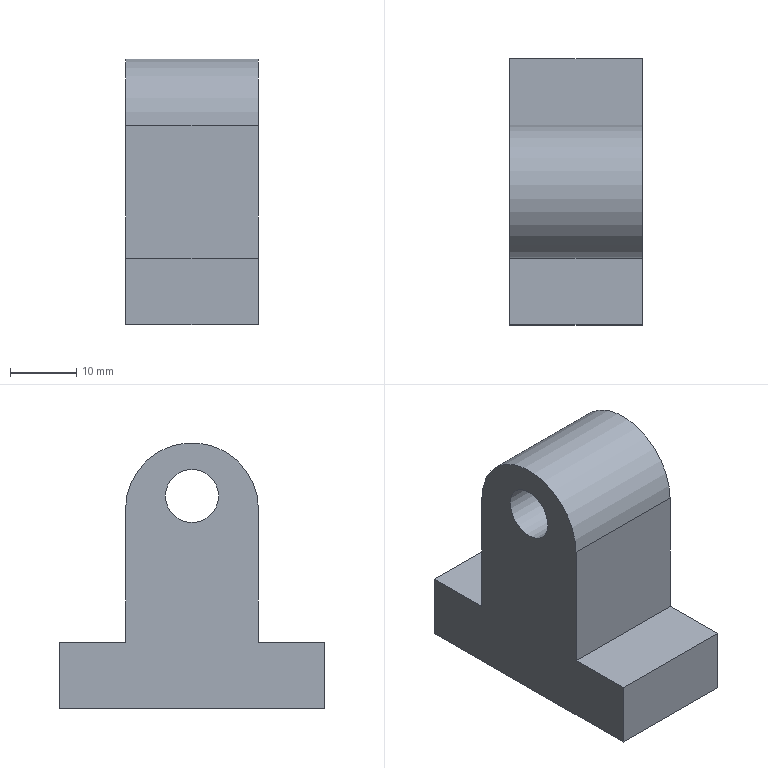Component | NX | T_SLIDER | 1 solid | 11 faces | box 20 x 40 x 40 mm | volume 18136 mm3 | plane 9 | cylinder 2 | commonest cylinder face diameters 20 x1 8 x1
STEP:
#1=CARTESIAN_POINT('',(0.,0.,0.));
#2=DIRECTION('',(0.,0.,1.));
#3=DIRECTION('',(1.,0.,0.));
#4=AXIS2_PLACEMENT_3D('',#1,#2,#3);
#5=CARTESIAN_POINT('',(-4.,-20.,10.));
#6=VERTEX_POINT('',#5);
#7=CARTESIAN_POINT('',(-4.,-20.,0.));
#8=VERTEX_POINT('',#7);
#9=CARTESIAN_POINT('',(-4.,-20.,10.));
#10=DIRECTION('',(0.,0.,-1.));
#11=VECTOR('',#10,1.);
#12=LINE('',#9,#11);
#13=CARTESIAN_POINT('',(16.,-20.,10.));
#14=DIRECTION('',(0.,1.,0.));
#15=DIRECTION('',(0.,-0.,1.));
#16=AXIS2_PLACEMENT_3D('',#13,#14,#15);
#17=PLANE('',#16);
#18=CARTESIAN_POINT('',(0.,-20.));
#19=DIRECTION('',(-1.,0.));
#20=VECTOR('',#19,1.);
#21=LINE('',#18,#20);
#22=(GEOMETRIC_REPRESENTATION_CONTEXT(2)PARAMETRIC_REPRESENTATION_CONTEXT()REPRESENTATION_CONTEXT('',''));
#23=DEFINITIONAL_REPRESENTATION('',(#21),#22);
#24=PCURVE('',#17,#23);
#25=CARTESIAN_POINT('',(-4.,-0.,30.));
#26=DIRECTION('',(1.,0.,0.));
#27=DIRECTION('',(0.,0.,-1.));
#28=AXIS2_PLACEMENT_3D('',#25,#26,#27);
#29=PLANE('',#28);
#30=CARTESIAN_POINT('',(20.,-20.));
#31=DIRECTION('',(1.,0.));
#32=VECTOR('',#31,1.);
#33=LINE('',#30,#32);
#34=(GEOMETRIC_REPRESENTATION_CONTEXT(2)PARAMETRIC_REPRESENTATION_CONTEXT()REPRESENTATION_CONTEXT('',''));
#35=DEFINITIONAL_REPRESENTATION('',(#33),#34);
#36=PCURVE('',#29,#35);
#37=SURFACE_CURVE('',#12,(#24,#36),.PCURVE_S1.);
#38=EDGE_CURVE('',#6,#8,#37,.T.);
#39=ORIENTED_EDGE('',*,*,#38,.T.);
#40=CARTESIAN_POINT('',(16.,-20.,0.));
#41=VERTEX_POINT('',#40);
#42=CARTESIAN_POINT('',(16.,-20.,0.));
#43=DIRECTION('',(-1.,0.,0.));
#44=VECTOR('',#43,1.);
#45=LINE('',#42,#44);
#46=CARTESIAN_POINT('',(-10.,0.));
#47=DIRECTION('',(0.,-1.));
#48=VECTOR('',#47,1.);
#49=LINE('',#46,#48);
#50=(GEOMETRIC_REPRESENTATION_CONTEXT(2)PARAMETRIC_REPRESENTATION_CONTEXT()REPRESENTATION_CONTEXT('',''));
#51=DEFINITIONAL_REPRESENTATION('',(#49),#50);
#52=PCURVE('',#17,#51);
#53=CARTESIAN_POINT('',(16.,-20.,0.));
#54=DIRECTION('',(0.,0.,1.));
#55=DIRECTION('',(1.,0.,0.));
#56=AXIS2_PLACEMENT_3D('',#53,#54,#55);
#57=PLANE('',#56);
#58=CARTESIAN_POINT('',(0.,0.));
#59=DIRECTION('',(-1.,0.));
#60=VECTOR('',#59,1.);
#61=LINE('',#58,#60);
#62=(GEOMETRIC_REPRESENTATION_CONTEXT(2)PARAMETRIC_REPRESENTATION_CONTEXT()REPRESENTATION_CONTEXT('',''));
#63=DEFINITIONAL_REPRESENTATION('',(#61),#62);
#64=PCURVE('',#57,#63);
#65=SURFACE_CURVE('',#45,(#52,#64),.PCURVE_S1.);
#66=EDGE_CURVE('',#41,#8,#65,.T.);
#67=ORIENTED_EDGE('',*,*,#66,.F.);
#68=CARTESIAN_POINT('',(16.,-20.,10.));
#69=VERTEX_POINT('',#68);
#70=CARTESIAN_POINT('',(16.,-20.,10.));
#71=DIRECTION('',(0.,0.,-1.));
#72=VECTOR('',#71,1.);
#73=LINE('',#70,#72);
#74=CARTESIAN_POINT('',(0.,0.));
#75=DIRECTION('',(-1.,0.));
#76=VECTOR('',#75,1.);
#77=LINE('',#74,#76);
#78=(GEOMETRIC_REPRESENTATION_CONTEXT(2)PARAMETRIC_REPRESENTATION_CONTEXT()REPRESENTATION_CONTEXT('',''));
#79=DEFINITIONAL_REPRESENTATION('',(#77),#78);
#80=PCURVE('',#17,#79);
#81=CARTESIAN_POINT('',(16.,-0.,30.));
#82=DIRECTION('',(1.,0.,0.));
#83=DIRECTION('',(0.,0.,-1.));
#84=AXIS2_PLACEMENT_3D('',#81,#82,#83);
#85=PLANE('',#84);
#86=CARTESIAN_POINT('',(20.,-20.));
#87=DIRECTION('',(1.,0.));
#88=VECTOR('',#87,1.);
#89=LINE('',#86,#88);
#90=(GEOMETRIC_REPRESENTATION_CONTEXT(2)PARAMETRIC_REPRESENTATION_CONTEXT()REPRESENTATION_CONTEXT('',''));
#91=DEFINITIONAL_REPRESENTATION('',(#89),#90);
#92=PCURVE('',#85,#91);
#93=SURFACE_CURVE('',#73,(#80,#92),.PCURVE_S1.);
#94=EDGE_CURVE('',#69,#41,#93,.T.);
#95=ORIENTED_EDGE('',*,*,#94,.F.);
#96=CARTESIAN_POINT('',(16.,-20.,10.));
#97=DIRECTION('',(-1.,0.,0.));
#98=VECTOR('',#97,1.);
#99=LINE('',#96,#98);
#100=CARTESIAN_POINT('',(0.,0.));
#101=DIRECTION('',(0.,-1.));
#102=VECTOR('',#101,1.);
#103=LINE('',#100,#102);
#104=(GEOMETRIC_REPRESENTATION_CONTEXT(2)PARAMETRIC_REPRESENTATION_CONTEXT()REPRESENTATION_CONTEXT('',''));
#105=DEFINITIONAL_REPRESENTATION('',(#103),#104);
#106=PCURVE('',#17,#105);
#107=CARTESIAN_POINT('',(16.,-10.,10.));
#108=DIRECTION('',(0.,0.,-1.));
#109=DIRECTION('',(-1.,0.,0.));
#110=AXIS2_PLACEMENT_3D('',#107,#108,#109);
#111=PLANE('',#110);
#112=CARTESIAN_POINT('',(0.,-10.));
#113=DIRECTION('',(1.,0.));
#114=VECTOR('',#113,1.);
#115=LINE('',#112,#114);
#116=(GEOMETRIC_REPRESENTATION_CONTEXT(2)PARAMETRIC_REPRESENTATION_CONTEXT()REPRESENTATION_CONTEXT('',''));
#117=DEFINITIONAL_REPRESENTATION('',(#115),#116);
#118=PCURVE('',#111,#117);
#119=SURFACE_CURVE('',#99,(#106,#118),.PCURVE_S1.);
#120=EDGE_CURVE('',#69,#6,#119,.T.);
#121=ORIENTED_EDGE('',*,*,#120,.T.);
#122=EDGE_LOOP('',(#39,#67,#95,#121));
#123=FACE_BOUND('',#122,.T.);
#124=ADVANCED_FACE('',(#123),#17,.F.);
#125=CARTESIAN_POINT('',(-4.,20.,0.));
#126=VERTEX_POINT('',#125);
#127=CARTESIAN_POINT('',(-4.,-20.,0.));
#128=DIRECTION('',(0.,1.,0.));
#129=VECTOR('',#128,1.);
#130=LINE('',#127,#129);
#131=CARTESIAN_POINT('',(-20.,0.));
#132=DIRECTION('',(0.,1.));
#133=VECTOR('',#132,1.);
#134=LINE('',#131,#133);
#135=(GEOMETRIC_REPRESENTATION_CONTEXT(2)PARAMETRIC_REPRESENTATION_CONTEXT()REPRESENTATION_CONTEXT('',''));
#136=DEFINITIONAL_REPRESENTATION('',(#134),#135);
#137=PCURVE('',#57,#136);
#138=CARTESIAN_POINT('',(30.,-20.));
#139=DIRECTION('',(0.,1.));
#140=VECTOR('',#139,1.);
#141=LINE('',#138,#140);
#142=(GEOMETRIC_REPRESENTATION_CONTEXT(2)PARAMETRIC_REPRESENTATION_CONTEXT()REPRESENTATION_CONTEXT('',''));
#143=DEFINITIONAL_REPRESENTATION('',(#141),#142);
#144=PCURVE('',#29,#143);
#145=SURFACE_CURVE('',#130,(#137,#144),.PCURVE_S1.);
#146=EDGE_CURVE('',#8,#126,#145,.T.);
#147=ORIENTED_EDGE('',*,*,#146,.T.);
#148=CARTESIAN_POINT('',(16.,20.,0.));
#149=VERTEX_POINT('',#148);
#150=CARTESIAN_POINT('',(16.,20.,0.));
#151=DIRECTION('',(-1.,0.,0.));
#152=VECTOR('',#151,1.);
#153=LINE('',#150,#152);
#154=CARTESIAN_POINT('',(0.,40.));
#155=DIRECTION('',(-1.,0.));
#156=VECTOR('',#155,1.);
#157=LINE('',#154,#156);
#158=(GEOMETRIC_REPRESENTATION_CONTEXT(2)PARAMETRIC_REPRESENTATION_CONTEXT()REPRESENTATION_CONTEXT('',''));
#159=DEFINITIONAL_REPRESENTATION('',(#157),#158);
#160=PCURVE('',#57,#159);
#161=CARTESIAN_POINT('',(16.,20.,0.));
#162=DIRECTION('',(0.,-1.,-0.));
#163=DIRECTION('',(0.,0.,-1.));
#164=AXIS2_PLACEMENT_3D('',#161,#162,#163);
#165=PLANE('',#164);
#166=CARTESIAN_POINT('',(0.,0.));
#167=DIRECTION('',(0.,-1.));
#168=VECTOR('',#167,1.);
#169=LINE('',#166,#168);
#170=(GEOMETRIC_REPRESENTATION_CONTEXT(2)PARAMETRIC_REPRESENTATION_CONTEXT()REPRESENTATION_CONTEXT('',''));
#171=DEFINITIONAL_REPRESENTATION('',(#169),#170);
#172=PCURVE('',#165,#171);
#173=SURFACE_CURVE('',#153,(#160,#172),.PCURVE_S1.);
#174=EDGE_CURVE('',#149,#126,#173,.T.);
#175=ORIENTED_EDGE('',*,*,#174,.F.);
#176=CARTESIAN_POINT('',(16.,-20.,0.));
#177=DIRECTION('',(0.,1.,0.));
#178=VECTOR('',#177,1.);
#179=LINE('',#176,#178);
#180=CARTESIAN_POINT('',(0.,0.));
#181=DIRECTION('',(0.,1.));
#182=VECTOR('',#181,1.);
#183=LINE('',#180,#182);
#184=(GEOMETRIC_REPRESENTATION_CONTEXT(2)PARAMETRIC_REPRESENTATION_CONTEXT()REPRESENTATION_CONTEXT('',''));
#185=DEFINITIONAL_REPRESENTATION('',(#183),#184);
#186=PCURVE('',#57,#185);
#187=CARTESIAN_POINT('',(30.,-20.));
#188=DIRECTION('',(0.,1.));
#189=VECTOR('',#188,1.);
#190=LINE('',#187,#189);
#191=(GEOMETRIC_REPRESENTATION_CONTEXT(2)PARAMETRIC_REPRESENTATION_CONTEXT()REPRESENTATION_CONTEXT('',''));
#192=DEFINITIONAL_REPRESENTATION('',(#190),#191);
#193=PCURVE('',#85,#192);
#194=SURFACE_CURVE('',#179,(#186,#193),.PCURVE_S1.);
#195=EDGE_CURVE('',#41,#149,#194,.T.);
#196=ORIENTED_EDGE('',*,*,#195,.F.);
#197=ORIENTED_EDGE('',*,*,#66,.T.);
#198=EDGE_LOOP('',(#147,#175,#196,#197));
#199=FACE_BOUND('',#198,.T.);
#200=ADVANCED_FACE('',(#199),#57,.F.);
#201=CARTESIAN_POINT('',(-4.,20.,10.));
#202=VERTEX_POINT('',#201);
#203=CARTESIAN_POINT('',(-4.,20.,0.));
#204=DIRECTION('',(0.,-0.,1.));
#205=VECTOR('',#204,1.);
#206=LINE('',#203,#205);
#207=CARTESIAN_POINT('',(0.,-20.));
#208=DIRECTION('',(-1.,0.));
#209=VECTOR('',#208,1.);
#210=LINE('',#207,#209);
#211=(GEOMETRIC_REPRESENTATION_CONTEXT(2)PARAMETRIC_REPRESENTATION_CONTEXT()REPRESENTATION_CONTEXT('',''));
#212=DEFINITIONAL_REPRESENTATION('',(#210),#211);
#213=PCURVE('',#165,#212);
#214=CARTESIAN_POINT('',(30.,20.));
#215=DIRECTION('',(-1.,-0.));
#216=VECTOR('',#215,1.);
#217=LINE('',#214,#216);
#218=(GEOMETRIC_REPRESENTATION_CONTEXT(2)PARAMETRIC_REPRESENTATION_CONTEXT()REPRESENTATION_CONTEXT('',''));
#219=DEFINITIONAL_REPRESENTATION('',(#217),#218);
#220=PCURVE('',#29,#219);
#221=SURFACE_CURVE('',#206,(#213,#220),.PCURVE_S1.);
#222=EDGE_CURVE('',#126,#202,#221,.T.);
#223=ORIENTED_EDGE('',*,*,#222,.T.);
#224=CARTESIAN_POINT('',(16.,20.,10.));
#225=VERTEX_POINT('',#224);
#226=CARTESIAN_POINT('',(16.,20.,10.));
#227=DIRECTION('',(-1.,0.,0.));
#228=VECTOR('',#227,1.);
#229=LINE('',#226,#228);
#230=CARTESIAN_POINT('',(-10.,0.));
#231=DIRECTION('',(0.,-1.));
#232=VECTOR('',#231,1.);
#233=LINE('',#230,#232);
#234=(GEOMETRIC_REPRESENTATION_CONTEXT(2)PARAMETRIC_REPRESENTATION_CONTEXT()REPRESENTATION_CONTEXT('',''));
#235=DEFINITIONAL_REPRESENTATION('',(#233),#234);
#236=PCURVE('',#165,#235);
#237=CARTESIAN_POINT('',(16.,20.,10.));
#238=DIRECTION('',(0.,0.,-1.));
#239=DIRECTION('',(-1.,0.,0.));
#240=AXIS2_PLACEMENT_3D('',#237,#238,#239);
#241=PLANE('',#240);
#242=CARTESIAN_POINT('',(0.,0.));
#243=DIRECTION('',(1.,0.));
#244=VECTOR('',#243,1.);
#245=LINE('',#242,#244);
#246=(GEOMETRIC_REPRESENTATION_CONTEXT(2)PARAMETRIC_REPRESENTATION_CONTEXT()REPRESENTATION_CONTEXT('',''));
#247=DEFINITIONAL_REPRESENTATION('',(#245),#246);
#248=PCURVE('',#241,#247);
#249=SURFACE_CURVE('',#229,(#236,#248),.PCURVE_S1.);
#250=EDGE_CURVE('',#225,#202,#249,.T.);
#251=ORIENTED_EDGE('',*,*,#250,.F.);
#252=CARTESIAN_POINT('',(16.,20.,0.));
#253=DIRECTION('',(0.,-0.,1.));
#254=VECTOR('',#253,1.);
#255=LINE('',#252,#254);
#256=CARTESIAN_POINT('',(0.,0.));
#257=DIRECTION('',(-1.,0.));
#258=VECTOR('',#257,1.);
#259=LINE('',#256,#258);
#260=(GEOMETRIC_REPRESENTATION_CONTEXT(2)PARAMETRIC_REPRESENTATION_CONTEXT()REPRESENTATION_CONTEXT('',''));
#261=DEFINITIONAL_REPRESENTATION('',(#259),#260);
#262=PCURVE('',#165,#261);
#263=CARTESIAN_POINT('',(30.,20.));
#264=DIRECTION('',(-1.,-0.));
#265=VECTOR('',#264,1.);
#266=LINE('',#263,#265);
#267=(GEOMETRIC_REPRESENTATION_CONTEXT(2)PARAMETRIC_REPRESENTATION_CONTEXT()REPRESENTATION_CONTEXT('',''));
#268=DEFINITIONAL_REPRESENTATION('',(#266),#267);
#269=PCURVE('',#85,#268);
#270=SURFACE_CURVE('',#255,(#262,#269),.PCURVE_S1.);
#271=EDGE_CURVE('',#149,#225,#270,.T.);
#272=ORIENTED_EDGE('',*,*,#271,.F.);
#273=ORIENTED_EDGE('',*,*,#174,.T.);
#274=EDGE_LOOP('',(#223,#251,#272,#273));
#275=FACE_BOUND('',#274,.T.);
#276=ADVANCED_FACE('',(#275),#165,.F.);
#277=CARTESIAN_POINT('',(-4.,10.,10.));
#278=VERTEX_POINT('',#277);
#279=CARTESIAN_POINT('',(-4.,20.,10.));
#280=DIRECTION('',(0.,-1.,0.));
#281=VECTOR('',#280,1.);
#282=LINE('',#279,#281);
#283=CARTESIAN_POINT('',(20.,0.));
#284=DIRECTION('',(0.,-1.));
#285=VECTOR('',#284,1.);
#286=LINE('',#283,#285);
#287=(GEOMETRIC_REPRESENTATION_CONTEXT(2)PARAMETRIC_REPRESENTATION_CONTEXT()REPRESENTATION_CONTEXT('',''));
#288=DEFINITIONAL_REPRESENTATION('',(#286),#287);
#289=PCURVE('',#241,#288);
#290=CARTESIAN_POINT('',(20.,20.));
#291=DIRECTION('',(0.,-1.));
#292=VECTOR('',#291,1.);
#293=LINE('',#290,#292);
#294=(GEOMETRIC_REPRESENTATION_CONTEXT(2)PARAMETRIC_REPRESENTATION_CONTEXT()REPRESENTATION_CONTEXT('',''));
#295=DEFINITIONAL_REPRESENTATION('',(#293),#294);
#296=PCURVE('',#29,#295);
#297=SURFACE_CURVE('',#282,(#289,#296),.PCURVE_S1.);
#298=EDGE_CURVE('',#202,#278,#297,.T.);
#299=ORIENTED_EDGE('',*,*,#298,.T.);
#300=CARTESIAN_POINT('',(16.,10.,10.));
#301=VERTEX_POINT('',#300);
#302=CARTESIAN_POINT('',(16.,10.,10.));
#303=DIRECTION('',(-1.,0.,0.));
#304=VECTOR('',#303,1.);
#305=LINE('',#302,#304);
#306=CARTESIAN_POINT('',(0.,-10.));
#307=DIRECTION('',(1.,0.));
#308=VECTOR('',#307,1.);
#309=LINE('',#306,#308);
#310=(GEOMETRIC_REPRESENTATION_CONTEXT(2)PARAMETRIC_REPRESENTATION_CONTEXT()REPRESENTATION_CONTEXT('',''));
#311=DEFINITIONAL_REPRESENTATION('',(#309),#310);
#312=PCURVE('',#241,#311);
#313=CARTESIAN_POINT('',(16.,10.,10.));
#314=DIRECTION('',(0.,-1.,-0.));
#315=DIRECTION('',(0.,0.,-1.));
#316=AXIS2_PLACEMENT_3D('',#313,#314,#315);
#317=PLANE('',#316);
#318=CARTESIAN_POINT('',(0.,0.));
#319=DIRECTION('',(0.,-1.));
#320=VECTOR('',#319,1.);
#321=LINE('',#318,#320);
#322=(GEOMETRIC_REPRESENTATION_CONTEXT(2)PARAMETRIC_REPRESENTATION_CONTEXT()REPRESENTATION_CONTEXT('',''));
#323=DEFINITIONAL_REPRESENTATION('',(#321),#322);
#324=PCURVE('',#317,#323);
#325=SURFACE_CURVE('',#305,(#312,#324),.PCURVE_S1.);
#326=EDGE_CURVE('',#301,#278,#325,.T.);
#327=ORIENTED_EDGE('',*,*,#326,.F.);
#328=CARTESIAN_POINT('',(16.,20.,10.));
#329=DIRECTION('',(0.,-1.,0.));
#330=VECTOR('',#329,1.);
#331=LINE('',#328,#330);
#332=CARTESIAN_POINT('',(0.,0.));
#333=DIRECTION('',(0.,-1.));
#334=VECTOR('',#333,1.);
#335=LINE('',#332,#334);
#336=(GEOMETRIC_REPRESENTATION_CONTEXT(2)PARAMETRIC_REPRESENTATION_CONTEXT()REPRESENTATION_CONTEXT('',''));
#337=DEFINITIONAL_REPRESENTATION('',(#335),#336);
#338=PCURVE('',#241,#337);
#339=CARTESIAN_POINT('',(20.,20.));
#340=DIRECTION('',(0.,-1.));
#341=VECTOR('',#340,1.);
#342=LINE('',#339,#341);
#343=(GEOMETRIC_REPRESENTATION_CONTEXT(2)PARAMETRIC_REPRESENTATION_CONTEXT()REPRESENTATION_CONTEXT('',''));
#344=DEFINITIONAL_REPRESENTATION('',(#342),#343);
#345=PCURVE('',#85,#344);
#346=SURFACE_CURVE('',#331,(#338,#345),.PCURVE_S1.);
#347=EDGE_CURVE('',#225,#301,#346,.T.);
#348=ORIENTED_EDGE('',*,*,#347,.F.);
#349=ORIENTED_EDGE('',*,*,#250,.T.);
#350=EDGE_LOOP('',(#299,#327,#348,#349));
#351=FACE_BOUND('',#350,.T.);
#352=ADVANCED_FACE('',(#351),#241,.F.);
#353=CARTESIAN_POINT('',(-4.,10.,30.));
#354=VERTEX_POINT('',#353);
#355=CARTESIAN_POINT('',(-4.,10.,10.));
#356=DIRECTION('',(0.,-0.,1.));
#357=VECTOR('',#356,1.);
#358=LINE('',#355,#357);
#359=CARTESIAN_POINT('',(0.,-20.));
#360=DIRECTION('',(-1.,0.));
#361=VECTOR('',#360,1.);
#362=LINE('',#359,#361);
#363=(GEOMETRIC_REPRESENTATION_CONTEXT(2)PARAMETRIC_REPRESENTATION_CONTEXT()REPRESENTATION_CONTEXT('',''));
#364=DEFINITIONAL_REPRESENTATION('',(#362),#363);
#365=PCURVE('',#317,#364);
#366=CARTESIAN_POINT('',(20.,10.));
#367=DIRECTION('',(-1.,-0.));
#368=VECTOR('',#367,1.);
#369=LINE('',#366,#368);
#370=(GEOMETRIC_REPRESENTATION_CONTEXT(2)PARAMETRIC_REPRESENTATION_CONTEXT()REPRESENTATION_CONTEXT('',''));
#371=DEFINITIONAL_REPRESENTATION('',(#369),#370);
#372=PCURVE('',#29,#371);
#373=SURFACE_CURVE('',#358,(#365,#372),.PCURVE_S1.);
#374=EDGE_CURVE('',#278,#354,#373,.T.);
#375=ORIENTED_EDGE('',*,*,#374,.T.);
#376=CARTESIAN_POINT('',(16.,10.,30.));
#377=VERTEX_POINT('',#376);
#378=CARTESIAN_POINT('',(16.,10.,30.));
#379=DIRECTION('',(-1.,0.,0.));
#380=VECTOR('',#379,1.);
#381=LINE('',#378,#380);
#382=CARTESIAN_POINT('',(-20.,0.));
#383=DIRECTION('',(0.,-1.));
#384=VECTOR('',#383,1.);
#385=LINE('',#382,#384);
#386=(GEOMETRIC_REPRESENTATION_CONTEXT(2)PARAMETRIC_REPRESENTATION_CONTEXT()REPRESENTATION_CONTEXT('',''));
#387=DEFINITIONAL_REPRESENTATION('',(#385),#386);
#388=PCURVE('',#317,#387);
#389=CARTESIAN_POINT('',(16.,-0.,30.));
#390=DIRECTION('',(-1.,0.,0.));
#391=DIRECTION('',(0.,0.,1.));
#392=AXIS2_PLACEMENT_3D('',#389,#390,#391);
#393=CYLINDRICAL_SURFACE('',#392,10.);
#394=CARTESIAN_POINT('',(1.571,0.));
#395=DIRECTION('',(0.,1.));
#396=VECTOR('',#395,1.);
#397=LINE('',#394,#396);
#398=(GEOMETRIC_REPRESENTATION_CONTEXT(2)PARAMETRIC_REPRESENTATION_CONTEXT()REPRESENTATION_CONTEXT('',''));
#399=DEFINITIONAL_REPRESENTATION('',(#397),#398);
#400=PCURVE('',#393,#399);
#401=SURFACE_CURVE('',#381,(#388,#400),.PCURVE_S1.);
#402=EDGE_CURVE('',#377,#354,#401,.T.);
#403=ORIENTED_EDGE('',*,*,#402,.F.);
#404=CARTESIAN_POINT('',(16.,10.,10.));
#405=DIRECTION('',(0.,-0.,1.));
#406=VECTOR('',#405,1.);
#407=LINE('',#404,#406);
#408=CARTESIAN_POINT('',(0.,0.));
#409=DIRECTION('',(-1.,0.));
#410=VECTOR('',#409,1.);
#411=LINE('',#408,#410);
#412=(GEOMETRIC_REPRESENTATION_CONTEXT(2)PARAMETRIC_REPRESENTATION_CONTEXT()REPRESENTATION_CONTEXT('',''));
#413=DEFINITIONAL_REPRESENTATION('',(#411),#412);
#414=PCURVE('',#317,#413);
#415=CARTESIAN_POINT('',(20.,10.));
#416=DIRECTION('',(-1.,-0.));
#417=VECTOR('',#416,1.);
#418=LINE('',#415,#417);
#419=(GEOMETRIC_REPRESENTATION_CONTEXT(2)PARAMETRIC_REPRESENTATION_CONTEXT()REPRESENTATION_CONTEXT('',''));
#420=DEFINITIONAL_REPRESENTATION('',(#418),#419);
#421=PCURVE('',#85,#420);
#422=SURFACE_CURVE('',#407,(#414,#421),.PCURVE_S1.);
#423=EDGE_CURVE('',#301,#377,#422,.T.);
#424=ORIENTED_EDGE('',*,*,#423,.F.);
#425=ORIENTED_EDGE('',*,*,#326,.T.);
#426=EDGE_LOOP('',(#375,#403,#424,#425));
#427=FACE_BOUND('',#426,.T.);
#428=ADVANCED_FACE('',(#427),#317,.F.);
#429=CARTESIAN_POINT('',(-4.,-10.,30.));
#430=VERTEX_POINT('',#429);
#431=CARTESIAN_POINT('',(-4.,-0.,30.));
#432=DIRECTION('',(1.,0.,0.));
#433=DIRECTION('',(0.,1.,0.));
#434=AXIS2_PLACEMENT_3D('',#431,#432,#433);
#435=CIRCLE('',#434,10.);
#436=CARTESIAN_POINT('',(1.571,20.));
#437=DIRECTION('',(-1.,0.));
#438=VECTOR('',#437,1.);
#439=LINE('',#436,#438);
#440=(GEOMETRIC_REPRESENTATION_CONTEXT(2)PARAMETRIC_REPRESENTATION_CONTEXT()REPRESENTATION_CONTEXT('',''));
#441=DEFINITIONAL_REPRESENTATION('',(#439),#440);
#442=PCURVE('',#393,#441);
#443=CARTESIAN_POINT('',(0.,0.));
#444=DIRECTION('',(0.,1.));
#445=AXIS2_PLACEMENT_2D('',#443,#444);
#446=CIRCLE('',#445,10.);
#447=(GEOMETRIC_REPRESENTATION_CONTEXT(2)PARAMETRIC_REPRESENTATION_CONTEXT()REPRESENTATION_CONTEXT('',''));
#448=DEFINITIONAL_REPRESENTATION('',(#446),#447);
#449=PCURVE('',#29,#448);
#450=SURFACE_CURVE('',#435,(#442,#449),.PCURVE_S1.);
#451=EDGE_CURVE('',#354,#430,#450,.T.);
#452=ORIENTED_EDGE('',*,*,#451,.T.);
#453=CARTESIAN_POINT('',(16.,-10.,30.));
#454=VERTEX_POINT('',#453);
#455=CARTESIAN_POINT('',(16.,-10.,30.));
#456=DIRECTION('',(-1.,0.,0.));
#457=VECTOR('',#456,1.);
#458=LINE('',#455,#457);
#459=CARTESIAN_POINT('',(-1.571,0.));
#460=DIRECTION('',(0.,1.));
#461=VECTOR('',#460,1.);
#462=LINE('',#459,#461);
#463=(GEOMETRIC_REPRESENTATION_CONTEXT(2)PARAMETRIC_REPRESENTATION_CONTEXT()REPRESENTATION_CONTEXT('',''));
#464=DEFINITIONAL_REPRESENTATION('',(#462),#463);
#465=PCURVE('',#393,#464);
#466=CARTESIAN_POINT('',(16.,-10.,30.));
#467=DIRECTION('',(0.,1.,0.));
#468=DIRECTION('',(0.,-0.,1.));
#469=AXIS2_PLACEMENT_3D('',#466,#467,#468);
#470=PLANE('',#469);
#471=CARTESIAN_POINT('',(0.,0.));
#472=DIRECTION('',(0.,-1.));
#473=VECTOR('',#472,1.);
#474=LINE('',#471,#473);
#475=(GEOMETRIC_REPRESENTATION_CONTEXT(2)PARAMETRIC_REPRESENTATION_CONTEXT()REPRESENTATION_CONTEXT('',''));
#476=DEFINITIONAL_REPRESENTATION('',(#474),#475);
#477=PCURVE('',#470,#476);
#478=SURFACE_CURVE('',#458,(#465,#477),.PCURVE_S1.);
#479=EDGE_CURVE('',#454,#430,#478,.T.);
#480=ORIENTED_EDGE('',*,*,#479,.F.);
#481=CARTESIAN_POINT('',(16.,-0.,30.));
#482=DIRECTION('',(1.,0.,0.));
#483=DIRECTION('',(0.,1.,0.));
#484=AXIS2_PLACEMENT_3D('',#481,#482,#483);
#485=CIRCLE('',#484,10.);
#486=CARTESIAN_POINT('',(1.571,0.));
#487=DIRECTION('',(-1.,0.));
#488=VECTOR('',#487,1.);
#489=LINE('',#486,#488);
#490=(GEOMETRIC_REPRESENTATION_CONTEXT(2)PARAMETRIC_REPRESENTATION_CONTEXT()REPRESENTATION_CONTEXT('',''));
#491=DEFINITIONAL_REPRESENTATION('',(#489),#490);
#492=PCURVE('',#393,#491);
#493=CARTESIAN_POINT('',(0.,0.));
#494=DIRECTION('',(0.,1.));
#495=AXIS2_PLACEMENT_2D('',#493,#494);
#496=CIRCLE('',#495,10.);
#497=(GEOMETRIC_REPRESENTATION_CONTEXT(2)PARAMETRIC_REPRESENTATION_CONTEXT()REPRESENTATION_CONTEXT('',''));
#498=DEFINITIONAL_REPRESENTATION('',(#496),#497);
#499=PCURVE('',#85,#498);
#500=SURFACE_CURVE('',#485,(#492,#499),.PCURVE_S1.);
#501=EDGE_CURVE('',#377,#454,#500,.T.);
#502=ORIENTED_EDGE('',*,*,#501,.F.);
#503=ORIENTED_EDGE('',*,*,#402,.T.);
#504=EDGE_LOOP('',(#452,#480,#502,#503));
#505=FACE_BOUND('',#504,.T.);
#506=ADVANCED_FACE('',(#505),#393,.T.);
#507=CARTESIAN_POINT('',(-4.,-10.,10.));
#508=VERTEX_POINT('',#507);
#509=CARTESIAN_POINT('',(-4.,-10.,30.));
#510=DIRECTION('',(0.,0.,-1.));
#511=VECTOR('',#510,1.);
#512=LINE('',#509,#511);
#513=CARTESIAN_POINT('',(0.,-20.));
#514=DIRECTION('',(-1.,0.));
#515=VECTOR('',#514,1.);
#516=LINE('',#513,#515);
#517=(GEOMETRIC_REPRESENTATION_CONTEXT(2)PARAMETRIC_REPRESENTATION_CONTEXT()REPRESENTATION_CONTEXT('',''));
#518=DEFINITIONAL_REPRESENTATION('',(#516),#517);
#519=PCURVE('',#470,#518);
#520=CARTESIAN_POINT('',(0.,-10.));
#521=DIRECTION('',(1.,0.));
#522=VECTOR('',#521,1.);
#523=LINE('',#520,#522);
#524=(GEOMETRIC_REPRESENTATION_CONTEXT(2)PARAMETRIC_REPRESENTATION_CONTEXT()REPRESENTATION_CONTEXT('',''));
#525=DEFINITIONAL_REPRESENTATION('',(#523),#524);
#526=PCURVE('',#29,#525);
#527=SURFACE_CURVE('',#512,(#519,#526),.PCURVE_S1.);
#528=EDGE_CURVE('',#430,#508,#527,.T.);
#529=ORIENTED_EDGE('',*,*,#528,.T.);
#530=CARTESIAN_POINT('',(16.,-10.,10.));
#531=VERTEX_POINT('',#530);
#532=CARTESIAN_POINT('',(16.,-10.,10.));
#533=DIRECTION('',(-1.,0.,0.));
#534=VECTOR('',#533,1.);
#535=LINE('',#532,#534);
#536=CARTESIAN_POINT('',(-20.,0.));
#537=DIRECTION('',(0.,-1.));
#538=VECTOR('',#537,1.);
#539=LINE('',#536,#538);
#540=(GEOMETRIC_REPRESENTATION_CONTEXT(2)PARAMETRIC_REPRESENTATION_CONTEXT()REPRESENTATION_CONTEXT('',''));
#541=DEFINITIONAL_REPRESENTATION('',(#539),#540);
#542=PCURVE('',#470,#541);
#543=CARTESIAN_POINT('',(0.,0.));
#544=DIRECTION('',(1.,0.));
#545=VECTOR('',#544,1.);
#546=LINE('',#543,#545);
#547=(GEOMETRIC_REPRESENTATION_CONTEXT(2)PARAMETRIC_REPRESENTATION_CONTEXT()REPRESENTATION_CONTEXT('',''));
#548=DEFINITIONAL_REPRESENTATION('',(#546),#547);
#549=PCURVE('',#111,#548);
#550=SURFACE_CURVE('',#535,(#542,#549),.PCURVE_S1.);
#551=EDGE_CURVE('',#531,#508,#550,.T.);
#552=ORIENTED_EDGE('',*,*,#551,.F.);
#553=CARTESIAN_POINT('',(16.,-10.,30.));
#554=DIRECTION('',(0.,0.,-1.));
#555=VECTOR('',#554,1.);
#556=LINE('',#553,#555);
#557=CARTESIAN_POINT('',(0.,0.));
#558=DIRECTION('',(-1.,0.));
#559=VECTOR('',#558,1.);
#560=LINE('',#557,#559);
#561=(GEOMETRIC_REPRESENTATION_CONTEXT(2)PARAMETRIC_REPRESENTATION_CONTEXT()REPRESENTATION_CONTEXT('',''));
#562=DEFINITIONAL_REPRESENTATION('',(#560),#561);
#563=PCURVE('',#470,#562);
#564=CARTESIAN_POINT('',(0.,-10.));
#565=DIRECTION('',(1.,0.));
#566=VECTOR('',#565,1.);
#567=LINE('',#564,#566);
#568=(GEOMETRIC_REPRESENTATION_CONTEXT(2)PARAMETRIC_REPRESENTATION_CONTEXT()REPRESENTATION_CONTEXT('',''));
#569=DEFINITIONAL_REPRESENTATION('',(#567),#568);
#570=PCURVE('',#85,#569);
#571=SURFACE_CURVE('',#556,(#563,#570),.PCURVE_S1.);
#572=EDGE_CURVE('',#454,#531,#571,.T.);
#573=ORIENTED_EDGE('',*,*,#572,.F.);
#574=ORIENTED_EDGE('',*,*,#479,.T.);
#575=EDGE_LOOP('',(#529,#552,#573,#574));
#576=FACE_BOUND('',#575,.T.);
#577=ADVANCED_FACE('',(#576),#470,.F.);
#578=CARTESIAN_POINT('',(-4.,-10.,10.));
#579=DIRECTION('',(0.,-1.,0.));
#580=VECTOR('',#579,1.);
#581=LINE('',#578,#580);
#582=CARTESIAN_POINT('',(20.,0.));
#583=DIRECTION('',(0.,-1.));
#584=VECTOR('',#583,1.);
#585=LINE('',#582,#584);
#586=(GEOMETRIC_REPRESENTATION_CONTEXT(2)PARAMETRIC_REPRESENTATION_CONTEXT()REPRESENTATION_CONTEXT('',''));
#587=DEFINITIONAL_REPRESENTATION('',(#585),#586);
#588=PCURVE('',#111,#587);
#589=CARTESIAN_POINT('',(20.,-10.));
#590=DIRECTION('',(0.,-1.));
#591=VECTOR('',#590,1.);
#592=LINE('',#589,#591);
#593=(GEOMETRIC_REPRESENTATION_CONTEXT(2)PARAMETRIC_REPRESENTATION_CONTEXT()REPRESENTATION_CONTEXT('',''));
#594=DEFINITIONAL_REPRESENTATION('',(#592),#593);
#595=PCURVE('',#29,#594);
#596=SURFACE_CURVE('',#581,(#588,#595),.PCURVE_S1.);
#597=EDGE_CURVE('',#508,#6,#596,.T.);
#598=ORIENTED_EDGE('',*,*,#597,.T.);
#599=ORIENTED_EDGE('',*,*,#120,.F.);
#600=CARTESIAN_POINT('',(16.,-10.,10.));
#601=DIRECTION('',(0.,-1.,0.));
#602=VECTOR('',#601,1.);
#603=LINE('',#600,#602);
#604=CARTESIAN_POINT('',(0.,0.));
#605=DIRECTION('',(0.,-1.));
#606=VECTOR('',#605,1.);
#607=LINE('',#604,#606);
#608=(GEOMETRIC_REPRESENTATION_CONTEXT(2)PARAMETRIC_REPRESENTATION_CONTEXT()REPRESENTATION_CONTEXT('',''));
#609=DEFINITIONAL_REPRESENTATION('',(#607),#608);
#610=PCURVE('',#111,#609);
#611=CARTESIAN_POINT('',(20.,-10.));
#612=DIRECTION('',(0.,-1.));
#613=VECTOR('',#612,1.);
#614=LINE('',#611,#613);
#615=(GEOMETRIC_REPRESENTATION_CONTEXT(2)PARAMETRIC_REPRESENTATION_CONTEXT()REPRESENTATION_CONTEXT('',''));
#616=DEFINITIONAL_REPRESENTATION('',(#614),#615);
#617=PCURVE('',#85,#616);
#618=SURFACE_CURVE('',#603,(#610,#617),.PCURVE_S1.);
#619=EDGE_CURVE('',#531,#69,#618,.T.);
#620=ORIENTED_EDGE('',*,*,#619,.F.);
#621=ORIENTED_EDGE('',*,*,#551,.T.);
#622=EDGE_LOOP('',(#598,#599,#620,#621));
#623=FACE_BOUND('',#622,.T.);
#624=ADVANCED_FACE('',(#623),#111,.F.);
#625=CARTESIAN_POINT('',(16.,4.,32.));
#626=VERTEX_POINT('',#625);
#627=CARTESIAN_POINT('',(16.,-0.,32.));
#628=DIRECTION('',(1.,0.,0.));
#629=DIRECTION('',(0.,1.,0.));
#630=AXIS2_PLACEMENT_3D('',#627,#628,#629);
#631=CIRCLE('',#630,4.);
#632=CARTESIAN_POINT('',(16.,-0.,32.));
#633=DIRECTION('',(-1.,0.,0.));
#634=DIRECTION('',(0.,0.,1.));
#635=AXIS2_PLACEMENT_3D('',#632,#633,#634);
#636=CYLINDRICAL_SURFACE('',#635,4.);
#637=CARTESIAN_POINT('',(7.854,0.));
#638=DIRECTION('',(-1.,0.));
#639=VECTOR('',#638,1.);
#640=LINE('',#637,#639);
#641=(GEOMETRIC_REPRESENTATION_CONTEXT(2)PARAMETRIC_REPRESENTATION_CONTEXT()REPRESENTATION_CONTEXT('',''));
#642=DEFINITIONAL_REPRESENTATION('',(#640),#641);
#643=PCURVE('',#636,#642);
#644=CARTESIAN_POINT('',(-2.,0.));
#645=DIRECTION('',(0.,1.));
#646=AXIS2_PLACEMENT_2D('',#644,#645);
#647=CIRCLE('',#646,4.);
#648=(GEOMETRIC_REPRESENTATION_CONTEXT(2)PARAMETRIC_REPRESENTATION_CONTEXT()REPRESENTATION_CONTEXT('',''));
#649=DEFINITIONAL_REPRESENTATION('',(#647),#648);
#650=PCURVE('',#85,#649);
#651=SURFACE_CURVE('',#631,(#643,#650),.PCURVE_S1.);
#652=EDGE_CURVE('',#626,#626,#651,.T.);
#653=ORIENTED_EDGE('',*,*,#652,.F.);
#654=CARTESIAN_POINT('',(-4.,4.,32.));
#655=VERTEX_POINT('',#654);
#656=CARTESIAN_POINT('',(16.,4.,32.));
#657=CARTESIAN_POINT('',(-4.,4.,32.));
#658=B_SPLINE_CURVE_WITH_KNOTS('',1,(#656,#657),.UNSPECIFIED.,.F.,.F.,(2,2),(0.,20.),.PIECEWISE_BEZIER_KNOTS.);
#659=CARTESIAN_POINT('',(7.854,0.));
#660=DIRECTION('',(0.,1.));
#661=VECTOR('',#660,1.);
#662=LINE('',#659,#661);
#663=(GEOMETRIC_REPRESENTATION_CONTEXT(2)PARAMETRIC_REPRESENTATION_CONTEXT()REPRESENTATION_CONTEXT('',''));
#664=DEFINITIONAL_REPRESENTATION('',(#662),#663);
#665=PCURVE('',#636,#664);
#666=CARTESIAN_POINT('',(1.571,0.));
#667=DIRECTION('',(0.,1.));
#668=VECTOR('',#667,1.);
#669=LINE('',#666,#668);
#670=(GEOMETRIC_REPRESENTATION_CONTEXT(2)PARAMETRIC_REPRESENTATION_CONTEXT()REPRESENTATION_CONTEXT('',''));
#671=DEFINITIONAL_REPRESENTATION('',(#669),#670);
#672=PCURVE('',#636,#671);
#673=SEAM_CURVE('',#658,(#665,#672),.PCURVE_S1.);
#674=EDGE_CURVE('',#626,#655,#673,.T.);
#675=ORIENTED_EDGE('',*,*,#674,.T.);
#676=CARTESIAN_POINT('',(-4.,-0.,32.));
#677=DIRECTION('',(1.,0.,0.));
#678=DIRECTION('',(0.,1.,0.));
#679=AXIS2_PLACEMENT_3D('',#676,#677,#678);
#680=CIRCLE('',#679,4.);
#681=CARTESIAN_POINT('',(7.854,20.));
#682=DIRECTION('',(-1.,0.));
#683=VECTOR('',#682,1.);
#684=LINE('',#681,#683);
#685=(GEOMETRIC_REPRESENTATION_CONTEXT(2)PARAMETRIC_REPRESENTATION_CONTEXT()REPRESENTATION_CONTEXT('',''));
#686=DEFINITIONAL_REPRESENTATION('',(#684),#685);
#687=PCURVE('',#636,#686);
#688=CARTESIAN_POINT('',(-2.,0.));
#689=DIRECTION('',(0.,1.));
#690=AXIS2_PLACEMENT_2D('',#688,#689);
#691=CIRCLE('',#690,4.);
#692=(GEOMETRIC_REPRESENTATION_CONTEXT(2)PARAMETRIC_REPRESENTATION_CONTEXT()REPRESENTATION_CONTEXT('',''));
#693=DEFINITIONAL_REPRESENTATION('',(#691),#692);
#694=PCURVE('',#29,#693);
#695=SURFACE_CURVE('',#680,(#687,#694),.PCURVE_S1.);
#696=EDGE_CURVE('',#655,#655,#695,.T.);
#697=ORIENTED_EDGE('',*,*,#696,.T.);
#698=ORIENTED_EDGE('',*,*,#674,.F.);
#699=EDGE_LOOP('',(#653,#675,#697,#698));
#700=FACE_BOUND('',#699,.F.);
#701=ADVANCED_FACE('',(#700),#636,.F.);
#702=ORIENTED_EDGE('',*,*,#94,.T.);
#703=ORIENTED_EDGE('',*,*,#195,.T.);
#704=ORIENTED_EDGE('',*,*,#271,.T.);
#705=ORIENTED_EDGE('',*,*,#347,.T.);
#706=ORIENTED_EDGE('',*,*,#423,.T.);
#707=ORIENTED_EDGE('',*,*,#501,.T.);
#708=ORIENTED_EDGE('',*,*,#572,.T.);
#709=ORIENTED_EDGE('',*,*,#619,.T.);
#710=EDGE_LOOP('',(#702,#703,#704,#705,#706,#707,#708,#709));
#711=FACE_BOUND('',#710,.T.);
#712=ORIENTED_EDGE('',*,*,#652,.F.);
#713=EDGE_LOOP('',(#712));
#714=FACE_BOUND('',#713,.T.);
#715=ADVANCED_FACE('',(#711,#714),#85,.T.);
#716=ORIENTED_EDGE('',*,*,#38,.F.);
#717=ORIENTED_EDGE('',*,*,#597,.F.);
#718=ORIENTED_EDGE('',*,*,#528,.F.);
#719=ORIENTED_EDGE('',*,*,#451,.F.);
#720=ORIENTED_EDGE('',*,*,#374,.F.);
#721=ORIENTED_EDGE('',*,*,#298,.F.);
#722=ORIENTED_EDGE('',*,*,#222,.F.);
#723=ORIENTED_EDGE('',*,*,#146,.F.);
#724=EDGE_LOOP('',(#716,#717,#718,#719,#720,#721,#722,#723));
#725=FACE_BOUND('',#724,.T.);
#726=ORIENTED_EDGE('',*,*,#696,.T.);
#727=EDGE_LOOP('',(#726));
#728=FACE_BOUND('',#727,.T.);
#729=ADVANCED_FACE('',(#725,#728),#29,.F.);
#730=CLOSED_SHELL('',(#124,#200,#276,#352,#428,#506,#577,#624,#701,#715,#729));
#731=MANIFOLD_SOLID_BREP('',#730);
#732=(LENGTH_UNIT()NAMED_UNIT(*)SI_UNIT(.MILLI.,.METRE.));
#733=UNCERTAINTY_MEASURE_WITH_UNIT(LENGTH_MEASURE(0.000001),#732,'','');
#734=(NAMED_UNIT(*)PLANE_ANGLE_UNIT()SI_UNIT($,.RADIAN.));
#735=(NAMED_UNIT(*)SI_UNIT($,.STERADIAN.)SOLID_ANGLE_UNIT());
#736=(GEOMETRIC_REPRESENTATION_CONTEXT(3)GLOBAL_UNCERTAINTY_ASSIGNED_CONTEXT((#733))GLOBAL_UNIT_ASSIGNED_CONTEXT((#732,#734,#735))REPRESENTATION_CONTEXT('',''));
#737=ADVANCED_BREP_SHAPE_REPRESENTATION('',(#4,#731),#736);